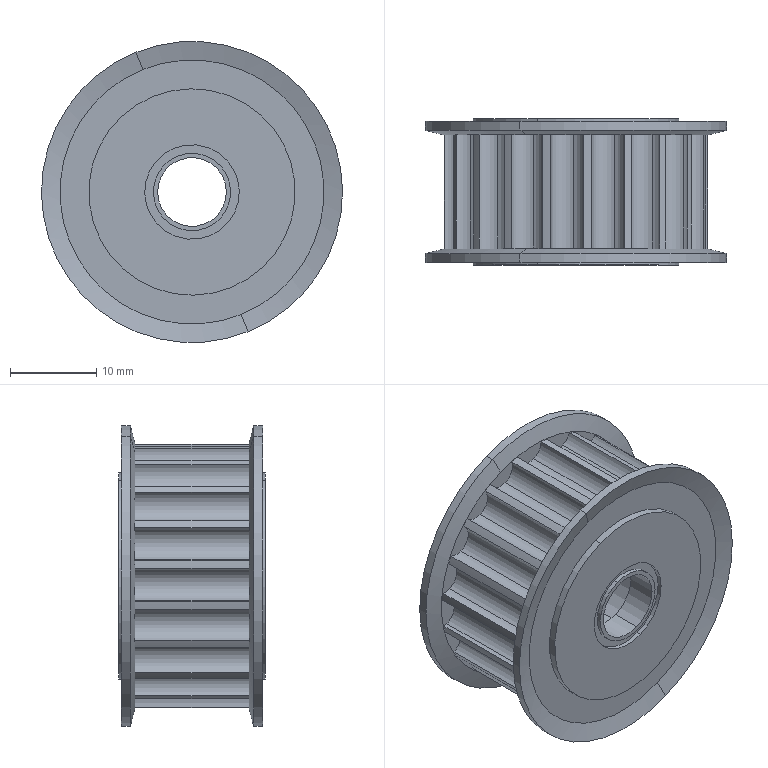Component | SolidWorks | ArcToothIdlerBearingTypeAtBothEnds[ST5GTD-20-12-Q]_ST5GTD-20-12-Q-1 | 1 solid | 91 faces | volume 9697 mm3 | cylinder 71 | plane 12 | cone 8 | commonest cylinder face diameters 3.86 x29 30.69 x20 11 x6 24 x4 9 x4 35 x4 8 x4